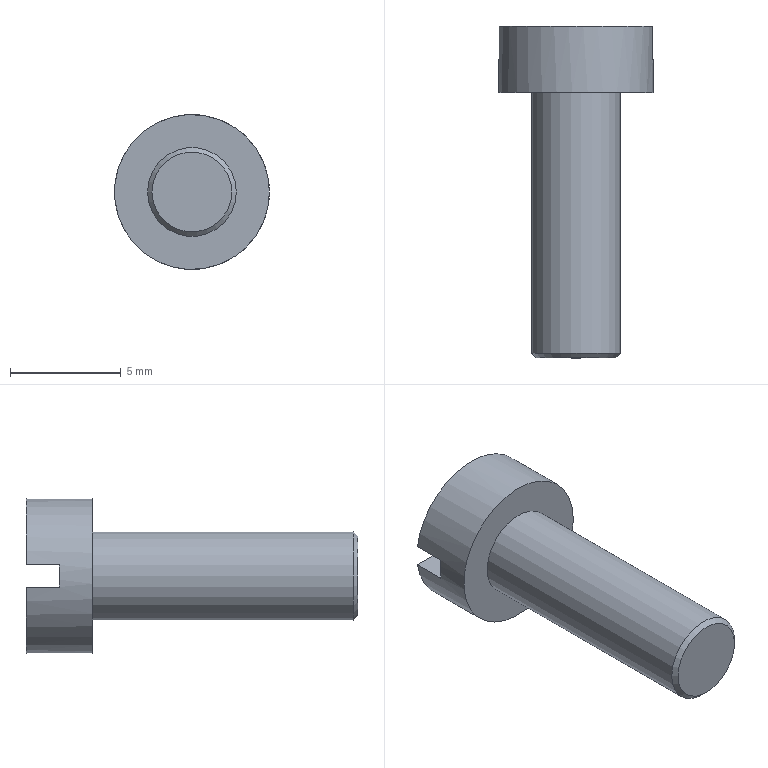Component | NX | SCREW_M4 | 1 solid | 10 faces | box 7 x 15 x 7 mm | volume 257 mm3 | plane 7 | cylinder 2 | cone 1 | commonest cylinder face diameters 7 x1 4.013 x1
STEP:
#1=CARTESIAN_POINT('',(0.,0.,0.));
#2=DIRECTION('',(0.,0.,1.));
#3=DIRECTION('',(1.,0.,0.));
#4=AXIS2_PLACEMENT_3D('',#1,#2,#3);
#5=CARTESIAN_POINT('',(23.036,8.,105.));
#6=VERTEX_POINT('',#5);
#7=CARTESIAN_POINT('',(29.964,8.,105.));
#8=VERTEX_POINT('',#7);
#9=CARTESIAN_POINT('',(26.5,8.,104.5));
#10=DIRECTION('',(0.,1.,0.));
#11=DIRECTION('',(1.,0.,0.));
#12=AXIS2_PLACEMENT_3D('',#9,#10,#11);
#13=CIRCLE('',#12,3.5);
#14=CARTESIAN_POINT('',(26.5,8.,104.5));
#15=DIRECTION('',(0.,1.,0.));
#16=DIRECTION('',(1.,0.,0.));
#17=AXIS2_PLACEMENT_3D('',#14,#15,#16);
#18=PLANE('',#17);
#19=CARTESIAN_POINT('',(0.,0.));
#20=DIRECTION('',(1.,0.));
#21=AXIS2_PLACEMENT_2D('',#19,#20);
#22=CIRCLE('',#21,3.5);
#23=(GEOMETRIC_REPRESENTATION_CONTEXT(2)PARAMETRIC_REPRESENTATION_CONTEXT()REPRESENTATION_CONTEXT('',''));
#24=DEFINITIONAL_REPRESENTATION('',(#22),#23);
#25=PCURVE('',#18,#24);
#26=CARTESIAN_POINT('',(26.5,5.,104.5));
#27=DIRECTION('',(0.,1.,0.));
#28=DIRECTION('',(1.,0.,0.));
#29=AXIS2_PLACEMENT_3D('',#26,#27,#28);
#30=CYLINDRICAL_SURFACE('',#29,3.5);
#31=CARTESIAN_POINT('',(0.,3.));
#32=DIRECTION('',(1.,0.));
#33=VECTOR('',#32,1.);
#34=LINE('',#31,#33);
#35=(GEOMETRIC_REPRESENTATION_CONTEXT(2)PARAMETRIC_REPRESENTATION_CONTEXT()REPRESENTATION_CONTEXT('',''));
#36=DEFINITIONAL_REPRESENTATION('',(#34),#35);
#37=PCURVE('',#30,#36);
#38=SURFACE_CURVE('',#13,(#25,#37),.PCURVE_S1.);
#39=EDGE_CURVE('',#6,#8,#38,.T.);
#40=ORIENTED_EDGE('',*,*,#39,.T.);
#41=CARTESIAN_POINT('',(30.786,8.,105.));
#42=DIRECTION('',(-1.,0.,0.));
#43=VECTOR('',#42,1.);
#44=LINE('',#41,#43);
#45=CARTESIAN_POINT('',(4.286,-0.5));
#46=DIRECTION('',(-1.,0.));
#47=VECTOR('',#46,1.);
#48=LINE('',#45,#47);
#49=(GEOMETRIC_REPRESENTATION_CONTEXT(2)PARAMETRIC_REPRESENTATION_CONTEXT()REPRESENTATION_CONTEXT('',''));
#50=DEFINITIONAL_REPRESENTATION('',(#48),#49);
#51=PCURVE('',#18,#50);
#52=CARTESIAN_POINT('',(30.786,6.5,105.));
#53=DIRECTION('',(0.,0.,-1.));
#54=DIRECTION('',(0.,1.,0.));
#55=AXIS2_PLACEMENT_3D('',#52,#53,#54);
#56=PLANE('',#55);
#57=CARTESIAN_POINT('',(1.5,0.));
#58=DIRECTION('',(0.,-1.));
#59=VECTOR('',#58,1.);
#60=LINE('',#57,#59);
#61=(GEOMETRIC_REPRESENTATION_CONTEXT(2)PARAMETRIC_REPRESENTATION_CONTEXT()REPRESENTATION_CONTEXT('',''));
#62=DEFINITIONAL_REPRESENTATION('',(#60),#61);
#63=PCURVE('',#56,#62);
#64=SURFACE_CURVE('',#44,(#51,#63),.PCURVE_S1.);
#65=EDGE_CURVE('',#8,#6,#64,.T.);
#66=ORIENTED_EDGE('',*,*,#65,.T.);
#67=EDGE_LOOP('',(#40,#66));
#68=FACE_BOUND('',#67,.T.);
#69=ADVANCED_FACE('',(#68),#18,.T.);
#70=CARTESIAN_POINT('',(29.964,8.,104.));
#71=VERTEX_POINT('',#70);
#72=CARTESIAN_POINT('',(23.036,8.,104.));
#73=VERTEX_POINT('',#72);
#74=CARTESIAN_POINT('',(26.5,8.,104.5));
#75=DIRECTION('',(0.,1.,0.));
#76=DIRECTION('',(1.,0.,0.));
#77=AXIS2_PLACEMENT_3D('',#74,#75,#76);
#78=CIRCLE('',#77,3.5);
#79=CARTESIAN_POINT('',(26.5,8.,104.5));
#80=DIRECTION('',(0.,1.,0.));
#81=DIRECTION('',(1.,0.,0.));
#82=AXIS2_PLACEMENT_3D('',#79,#80,#81);
#83=PLANE('',#82);
#84=CARTESIAN_POINT('',(0.,0.));
#85=DIRECTION('',(1.,0.));
#86=AXIS2_PLACEMENT_2D('',#84,#85);
#87=CIRCLE('',#86,3.5);
#88=(GEOMETRIC_REPRESENTATION_CONTEXT(2)PARAMETRIC_REPRESENTATION_CONTEXT()REPRESENTATION_CONTEXT('',''));
#89=DEFINITIONAL_REPRESENTATION('',(#87),#88);
#90=PCURVE('',#83,#89);
#91=CARTESIAN_POINT('',(0.,3.));
#92=DIRECTION('',(1.,0.));
#93=VECTOR('',#92,1.);
#94=LINE('',#91,#93);
#95=(GEOMETRIC_REPRESENTATION_CONTEXT(2)PARAMETRIC_REPRESENTATION_CONTEXT()REPRESENTATION_CONTEXT('',''));
#96=DEFINITIONAL_REPRESENTATION('',(#94),#95);
#97=PCURVE('',#30,#96);
#98=SURFACE_CURVE('',#78,(#90,#97),.PCURVE_S1.);
#99=EDGE_CURVE('',#71,#73,#98,.T.);
#100=ORIENTED_EDGE('',*,*,#99,.T.);
#101=CARTESIAN_POINT('',(22.214,8.,104.));
#102=DIRECTION('',(1.,0.,0.));
#103=VECTOR('',#102,1.);
#104=LINE('',#101,#103);
#105=CARTESIAN_POINT('',(-4.286,0.5));
#106=DIRECTION('',(1.,0.));
#107=VECTOR('',#106,1.);
#108=LINE('',#105,#107);
#109=(GEOMETRIC_REPRESENTATION_CONTEXT(2)PARAMETRIC_REPRESENTATION_CONTEXT()REPRESENTATION_CONTEXT('',''));
#110=DEFINITIONAL_REPRESENTATION('',(#108),#109);
#111=PCURVE('',#83,#110);
#112=CARTESIAN_POINT('',(22.214,6.5,104.));
#113=DIRECTION('',(0.,0.,1.));
#114=DIRECTION('',(0.,-1.,0.));
#115=AXIS2_PLACEMENT_3D('',#112,#113,#114);
#116=PLANE('',#115);
#117=CARTESIAN_POINT('',(-1.5,0.));
#118=DIRECTION('',(0.,1.));
#119=VECTOR('',#118,1.);
#120=LINE('',#117,#119);
#121=(GEOMETRIC_REPRESENTATION_CONTEXT(2)PARAMETRIC_REPRESENTATION_CONTEXT()REPRESENTATION_CONTEXT('',''));
#122=DEFINITIONAL_REPRESENTATION('',(#120),#121);
#123=PCURVE('',#116,#122);
#124=SURFACE_CURVE('',#104,(#111,#123),.PCURVE_S1.);
#125=EDGE_CURVE('',#73,#71,#124,.T.);
#126=ORIENTED_EDGE('',*,*,#125,.T.);
#127=EDGE_LOOP('',(#100,#126));
#128=FACE_BOUND('',#127,.T.);
#129=ADVANCED_FACE('',(#128),#83,.T.);
#130=CARTESIAN_POINT('',(30.,5.,104.5));
#131=VERTEX_POINT('',#130);
#132=CARTESIAN_POINT('',(26.5,5.,104.5));
#133=DIRECTION('',(0.,1.,0.));
#134=DIRECTION('',(1.,0.,0.));
#135=AXIS2_PLACEMENT_3D('',#132,#133,#134);
#136=CIRCLE('',#135,3.5);
#137=CARTESIAN_POINT('',(0.,0.));
#138=DIRECTION('',(1.,0.));
#139=VECTOR('',#138,1.);
#140=LINE('',#137,#139);
#141=(GEOMETRIC_REPRESENTATION_CONTEXT(2)PARAMETRIC_REPRESENTATION_CONTEXT()REPRESENTATION_CONTEXT('',''));
#142=DEFINITIONAL_REPRESENTATION('',(#140),#141);
#143=PCURVE('',#30,#142);
#144=CARTESIAN_POINT('',(26.5,5.,104.5));
#145=DIRECTION('',(0.,-1.,0.));
#146=DIRECTION('',(-1.,0.,0.));
#147=AXIS2_PLACEMENT_3D('',#144,#145,#146);
#148=PLANE('',#147);
#149=CARTESIAN_POINT('',(-3.5,0.));
#150=CARTESIAN_POINT('',(-3.5,6.062));
#151=CARTESIAN_POINT('',(1.75,3.031));
#152=CARTESIAN_POINT('',(7.,0.));
#153=CARTESIAN_POINT('',(1.75,-3.031));
#154=CARTESIAN_POINT('',(-3.5,-6.062));
#155=CARTESIAN_POINT('',(-3.5,0.));
#156=(BOUNDED_CURVE()B_SPLINE_CURVE(2,(#149,#150,#151,#152,#153,#154,#155),.UNSPECIFIED.,.T.,.F.)B_SPLINE_CURVE_WITH_KNOTS((1,2,2,2,2,1),(-2.094,0.,2.094,4.189,6.283,8.378),.UNSPECIFIED.)CURVE()GEOMETRIC_REPRESENTATION_ITEM()RATIONAL_B_SPLINE_CURVE((1.,0.5,1.,0.5,1.,0.5,1.))REPRESENTATION_ITEM(''));
#157=(GEOMETRIC_REPRESENTATION_CONTEXT(2)PARAMETRIC_REPRESENTATION_CONTEXT()REPRESENTATION_CONTEXT('',''));
#158=DEFINITIONAL_REPRESENTATION('',(#156),#157);
#159=PCURVE('',#148,#158);
#160=SURFACE_CURVE('',#136,(#143,#159),.PCURVE_S1.);
#161=EDGE_CURVE('',#131,#131,#160,.T.);
#162=ORIENTED_EDGE('',*,*,#161,.T.);
#163=CARTESIAN_POINT('',(30.,6.5,104.5));
#164=VERTEX_POINT('',#163);
#165=CARTESIAN_POINT('',(30.,5.,104.5));
#166=CARTESIAN_POINT('',(30.,6.5,104.5));
#167=B_SPLINE_CURVE_WITH_KNOTS('',1,(#165,#166),.UNSPECIFIED.,.F.,.F.,(2,2),(0.,1.5),.PIECEWISE_BEZIER_KNOTS.);
#168=CARTESIAN_POINT('',(6.283,0.));
#169=DIRECTION('',(0.,1.));
#170=VECTOR('',#169,1.);
#171=LINE('',#168,#170);
#172=(GEOMETRIC_REPRESENTATION_CONTEXT(2)PARAMETRIC_REPRESENTATION_CONTEXT()REPRESENTATION_CONTEXT('',''));
#173=DEFINITIONAL_REPRESENTATION('',(#171),#172);
#174=PCURVE('',#30,#173);
#175=CARTESIAN_POINT('',(0.,0.));
#176=DIRECTION('',(0.,1.));
#177=VECTOR('',#176,1.);
#178=LINE('',#175,#177);
#179=(GEOMETRIC_REPRESENTATION_CONTEXT(2)PARAMETRIC_REPRESENTATION_CONTEXT()REPRESENTATION_CONTEXT('',''));
#180=DEFINITIONAL_REPRESENTATION('',(#178),#179);
#181=PCURVE('',#30,#180);
#182=SEAM_CURVE('',#167,(#174,#181),.PCURVE_S1.);
#183=EDGE_CURVE('',#131,#164,#182,.T.);
#184=ORIENTED_EDGE('',*,*,#183,.T.);
#185=CARTESIAN_POINT('',(29.964,6.5,105.));
#186=VERTEX_POINT('',#185);
#187=CARTESIAN_POINT('',(26.5,6.5,104.5));
#188=DIRECTION('',(0.,1.,0.));
#189=DIRECTION('',(-1.,0.,0.));
#190=AXIS2_PLACEMENT_3D('',#187,#188,#189);
#191=CIRCLE('',#190,3.5);
#192=CARTESIAN_POINT('',(3.142,1.5));
#193=DIRECTION('',(1.,0.));
#194=VECTOR('',#193,1.);
#195=LINE('',#192,#194);
#196=(GEOMETRIC_REPRESENTATION_CONTEXT(2)PARAMETRIC_REPRESENTATION_CONTEXT()REPRESENTATION_CONTEXT('',''));
#197=DEFINITIONAL_REPRESENTATION('',(#195),#196);
#198=PCURVE('',#30,#197);
#199=CARTESIAN_POINT('',(26.5,6.5,104.5));
#200=DIRECTION('',(0.,-1.,0.));
#201=DIRECTION('',(-1.,0.,0.));
#202=AXIS2_PLACEMENT_3D('',#199,#200,#201);
#203=PLANE('',#202);
#204=CARTESIAN_POINT('',(3.5,0.));
#205=CARTESIAN_POINT('',(3.5,-6.062));
#206=CARTESIAN_POINT('',(-1.75,-3.031));
#207=CARTESIAN_POINT('',(-7.,-0.));
#208=CARTESIAN_POINT('',(-1.75,3.031));
#209=CARTESIAN_POINT('',(3.5,6.062));
#210=CARTESIAN_POINT('',(3.5,0.));
#211=(BOUNDED_CURVE()B_SPLINE_CURVE(2,(#204,#205,#206,#207,#208,#209,#210),.UNSPECIFIED.,.T.,.F.)B_SPLINE_CURVE_WITH_KNOTS((1,2,2,2,2,1),(-2.094,0.,2.094,4.189,6.283,8.378),.UNSPECIFIED.)CURVE()GEOMETRIC_REPRESENTATION_ITEM()RATIONAL_B_SPLINE_CURVE((1.,0.5,1.,0.5,1.,0.5,1.))REPRESENTATION_ITEM(''));
#212=(GEOMETRIC_REPRESENTATION_CONTEXT(2)PARAMETRIC_REPRESENTATION_CONTEXT()REPRESENTATION_CONTEXT('',''));
#213=DEFINITIONAL_REPRESENTATION('',(#211),#212);
#214=PCURVE('',#203,#213);
#215=SURFACE_CURVE('',#191,(#198,#214),.PCURVE_S1.);
#216=EDGE_CURVE('',#186,#164,#215,.T.);
#217=ORIENTED_EDGE('',*,*,#216,.F.);
#218=CARTESIAN_POINT('',(29.964,5.,105.));
#219=DIRECTION('',(0.,1.,0.));
#220=VECTOR('',#219,1.);
#221=LINE('',#218,#220);
#222=CARTESIAN_POINT('',(6.14,0.));
#223=DIRECTION('',(0.,1.));
#224=VECTOR('',#223,1.);
#225=LINE('',#222,#224);
#226=(GEOMETRIC_REPRESENTATION_CONTEXT(2)PARAMETRIC_REPRESENTATION_CONTEXT()REPRESENTATION_CONTEXT('',''));
#227=DEFINITIONAL_REPRESENTATION('',(#225),#226);
#228=PCURVE('',#30,#227);
#229=CARTESIAN_POINT('',(-1.5,-0.822));
#230=DIRECTION('',(1.,0.));
#231=VECTOR('',#230,1.);
#232=LINE('',#229,#231);
#233=(GEOMETRIC_REPRESENTATION_CONTEXT(2)PARAMETRIC_REPRESENTATION_CONTEXT()REPRESENTATION_CONTEXT('',''));
#234=DEFINITIONAL_REPRESENTATION('',(#232),#233);
#235=PCURVE('',#56,#234);
#236=SURFACE_CURVE('',#221,(#228,#235),.PCURVE_S1.);
#237=EDGE_CURVE('',#186,#8,#236,.T.);
#238=ORIENTED_EDGE('',*,*,#237,.T.);
#239=ORIENTED_EDGE('',*,*,#39,.F.);
#240=CARTESIAN_POINT('',(23.036,6.5,105.));
#241=VERTEX_POINT('',#240);
#242=CARTESIAN_POINT('',(23.036,5.,105.));
#243=DIRECTION('',(0.,-1.,0.));
#244=VECTOR('',#243,1.);
#245=LINE('',#242,#244);
#246=CARTESIAN_POINT('',(3.285,0.));
#247=DIRECTION('',(0.,-1.));
#248=VECTOR('',#247,1.);
#249=LINE('',#246,#248);
#250=(GEOMETRIC_REPRESENTATION_CONTEXT(2)PARAMETRIC_REPRESENTATION_CONTEXT()REPRESENTATION_CONTEXT('',''));
#251=DEFINITIONAL_REPRESENTATION('',(#249),#250);
#252=PCURVE('',#30,#251);
#253=CARTESIAN_POINT('',(-1.5,-7.75));
#254=DIRECTION('',(-1.,0.));
#255=VECTOR('',#254,1.);
#256=LINE('',#253,#255);
#257=(GEOMETRIC_REPRESENTATION_CONTEXT(2)PARAMETRIC_REPRESENTATION_CONTEXT()REPRESENTATION_CONTEXT('',''));
#258=DEFINITIONAL_REPRESENTATION('',(#256),#257);
#259=PCURVE('',#56,#258);
#260=SURFACE_CURVE('',#245,(#252,#259),.PCURVE_S1.);
#261=EDGE_CURVE('',#6,#241,#260,.T.);
#262=ORIENTED_EDGE('',*,*,#261,.T.);
#263=CARTESIAN_POINT('',(23.036,6.5,104.));
#264=VERTEX_POINT('',#263);
#265=CARTESIAN_POINT('',(26.5,6.5,104.5));
#266=DIRECTION('',(0.,1.,0.));
#267=DIRECTION('',(-1.,0.,0.));
#268=AXIS2_PLACEMENT_3D('',#265,#266,#267);
#269=CIRCLE('',#268,3.5);
#270=CARTESIAN_POINT('',(-3.142,1.5));
#271=DIRECTION('',(1.,0.));
#272=VECTOR('',#271,1.);
#273=LINE('',#270,#272);
#274=(GEOMETRIC_REPRESENTATION_CONTEXT(2)PARAMETRIC_REPRESENTATION_CONTEXT()REPRESENTATION_CONTEXT('',''));
#275=DEFINITIONAL_REPRESENTATION('',(#273),#274);
#276=PCURVE('',#30,#275);
#277=CARTESIAN_POINT('',(3.5,0.));
#278=CARTESIAN_POINT('',(3.5,-6.062));
#279=CARTESIAN_POINT('',(-1.75,-3.031));
#280=CARTESIAN_POINT('',(-7.,-0.));
#281=CARTESIAN_POINT('',(-1.75,3.031));
#282=CARTESIAN_POINT('',(3.5,6.062));
#283=CARTESIAN_POINT('',(3.5,0.));
#284=(BOUNDED_CURVE()B_SPLINE_CURVE(2,(#277,#278,#279,#280,#281,#282,#283),.UNSPECIFIED.,.T.,.F.)B_SPLINE_CURVE_WITH_KNOTS((1,2,2,2,2,1),(-2.094,0.,2.094,4.189,6.283,8.378),.UNSPECIFIED.)CURVE()GEOMETRIC_REPRESENTATION_ITEM()RATIONAL_B_SPLINE_CURVE((1.,0.5,1.,0.5,1.,0.5,1.))REPRESENTATION_ITEM(''));
#285=(GEOMETRIC_REPRESENTATION_CONTEXT(2)PARAMETRIC_REPRESENTATION_CONTEXT()REPRESENTATION_CONTEXT('',''));
#286=DEFINITIONAL_REPRESENTATION('',(#284),#285);
#287=PCURVE('',#203,#286);
#288=SURFACE_CURVE('',#269,(#276,#287),.PCURVE_S1.);
#289=EDGE_CURVE('',#264,#241,#288,.T.);
#290=ORIENTED_EDGE('',*,*,#289,.F.);
#291=CARTESIAN_POINT('',(23.036,5.,104.));
#292=DIRECTION('',(0.,1.,0.));
#293=VECTOR('',#292,1.);
#294=LINE('',#291,#293);
#295=CARTESIAN_POINT('',(2.998,0.));
#296=DIRECTION('',(0.,1.));
#297=VECTOR('',#296,1.);
#298=LINE('',#295,#297);
#299=(GEOMETRIC_REPRESENTATION_CONTEXT(2)PARAMETRIC_REPRESENTATION_CONTEXT()REPRESENTATION_CONTEXT('',''));
#300=DEFINITIONAL_REPRESENTATION('',(#298),#299);
#301=PCURVE('',#30,#300);
#302=CARTESIAN_POINT('',(1.5,0.822));
#303=DIRECTION('',(-1.,0.));
#304=VECTOR('',#303,1.);
#305=LINE('',#302,#304);
#306=(GEOMETRIC_REPRESENTATION_CONTEXT(2)PARAMETRIC_REPRESENTATION_CONTEXT()REPRESENTATION_CONTEXT('',''));
#307=DEFINITIONAL_REPRESENTATION('',(#305),#306);
#308=PCURVE('',#116,#307);
#309=SURFACE_CURVE('',#294,(#301,#308),.PCURVE_S1.);
#310=EDGE_CURVE('',#264,#73,#309,.T.);
#311=ORIENTED_EDGE('',*,*,#310,.T.);
#312=ORIENTED_EDGE('',*,*,#99,.F.);
#313=CARTESIAN_POINT('',(29.964,6.5,104.));
#314=VERTEX_POINT('',#313);
#315=CARTESIAN_POINT('',(29.964,5.,104.));
#316=DIRECTION('',(0.,-1.,0.));
#317=VECTOR('',#316,1.);
#318=LINE('',#315,#317);
#319=CARTESIAN_POINT('',(0.1433,0.));
#320=DIRECTION('',(0.,-1.));
#321=VECTOR('',#320,1.);
#322=LINE('',#319,#321);
#323=(GEOMETRIC_REPRESENTATION_CONTEXT(2)PARAMETRIC_REPRESENTATION_CONTEXT()REPRESENTATION_CONTEXT('',''));
#324=DEFINITIONAL_REPRESENTATION('',(#322),#323);
#325=PCURVE('',#30,#324);
#326=CARTESIAN_POINT('',(1.5,7.75));
#327=DIRECTION('',(1.,0.));
#328=VECTOR('',#327,1.);
#329=LINE('',#326,#328);
#330=(GEOMETRIC_REPRESENTATION_CONTEXT(2)PARAMETRIC_REPRESENTATION_CONTEXT()REPRESENTATION_CONTEXT('',''));
#331=DEFINITIONAL_REPRESENTATION('',(#329),#330);
#332=PCURVE('',#116,#331);
#333=SURFACE_CURVE('',#318,(#325,#332),.PCURVE_S1.);
#334=EDGE_CURVE('',#71,#314,#333,.T.);
#335=ORIENTED_EDGE('',*,*,#334,.T.);
#336=CARTESIAN_POINT('',(26.5,6.5,104.5));
#337=DIRECTION('',(0.,1.,0.));
#338=DIRECTION('',(-1.,0.,0.));
#339=AXIS2_PLACEMENT_3D('',#336,#337,#338);
#340=CIRCLE('',#339,3.5);
#341=CARTESIAN_POINT('',(-3.142,1.5));
#342=DIRECTION('',(1.,0.));
#343=VECTOR('',#342,1.);
#344=LINE('',#341,#343);
#345=(GEOMETRIC_REPRESENTATION_CONTEXT(2)PARAMETRIC_REPRESENTATION_CONTEXT()REPRESENTATION_CONTEXT('',''));
#346=DEFINITIONAL_REPRESENTATION('',(#344),#345);
#347=PCURVE('',#30,#346);
#348=CARTESIAN_POINT('',(3.5,0.));
#349=CARTESIAN_POINT('',(3.5,-6.062));
#350=CARTESIAN_POINT('',(-1.75,-3.031));
#351=CARTESIAN_POINT('',(-7.,-0.));
#352=CARTESIAN_POINT('',(-1.75,3.031));
#353=CARTESIAN_POINT('',(3.5,6.062));
#354=CARTESIAN_POINT('',(3.5,0.));
#355=(BOUNDED_CURVE()B_SPLINE_CURVE(2,(#348,#349,#350,#351,#352,#353,#354),.UNSPECIFIED.,.T.,.F.)B_SPLINE_CURVE_WITH_KNOTS((1,2,2,2,2,1),(-2.094,0.,2.094,4.189,6.283,8.378),.UNSPECIFIED.)CURVE()GEOMETRIC_REPRESENTATION_ITEM()RATIONAL_B_SPLINE_CURVE((1.,0.5,1.,0.5,1.,0.5,1.))REPRESENTATION_ITEM(''));
#356=(GEOMETRIC_REPRESENTATION_CONTEXT(2)PARAMETRIC_REPRESENTATION_CONTEXT()REPRESENTATION_CONTEXT('',''));
#357=DEFINITIONAL_REPRESENTATION('',(#355),#356);
#358=PCURVE('',#203,#357);
#359=SURFACE_CURVE('',#340,(#347,#358),.PCURVE_S1.);
#360=EDGE_CURVE('',#164,#314,#359,.T.);
#361=ORIENTED_EDGE('',*,*,#360,.F.);
#362=ORIENTED_EDGE('',*,*,#183,.F.);
#363=EDGE_LOOP('',(#162,#184,#217,#238,#239,#262,#290,#311,#312,#335,#361,#362));
#364=FACE_BOUND('',#363,.T.);
#365=ADVANCED_FACE('',(#364),#30,.T.);
#366=CARTESIAN_POINT('',(24.693,-7.,104.5));
#367=VERTEX_POINT('',#366);
#368=CARTESIAN_POINT('',(26.5,-7.,104.5));
#369=DIRECTION('',(0.,-1.,0.));
#370=DIRECTION('',(-1.,0.,0.));
#371=AXIS2_PLACEMENT_3D('',#368,#369,#370);
#372=CIRCLE('',#371,1.807);
#373=CARTESIAN_POINT('',(26.5,-7.,104.5));
#374=DIRECTION('',(0.,-1.,0.));
#375=DIRECTION('',(-1.,0.,0.));
#376=AXIS2_PLACEMENT_3D('',#373,#374,#375);
#377=PLANE('',#376);
#378=CARTESIAN_POINT('',(0.,0.));
#379=DIRECTION('',(1.,0.));
#380=AXIS2_PLACEMENT_2D('',#378,#379);
#381=CIRCLE('',#380,1.807);
#382=(GEOMETRIC_REPRESENTATION_CONTEXT(2)PARAMETRIC_REPRESENTATION_CONTEXT()REPRESENTATION_CONTEXT('',''));
#383=DEFINITIONAL_REPRESENTATION('',(#381),#382);
#384=PCURVE('',#377,#383);
#385=CARTESIAN_POINT('',(26.5,-6.8,104.5));
#386=DIRECTION('',(0.,1.,0.));
#387=DIRECTION('',(1.,0.,0.));
#388=AXIS2_PLACEMENT_3D('',#385,#386,#387);
#389=CONICAL_SURFACE('',#388,2.007,0.7854);
#390=CARTESIAN_POINT('',(9.425,-0.2));
#391=DIRECTION('',(-1.,0.));
#392=VECTOR('',#391,1.);
#393=LINE('',#390,#392);
#394=(GEOMETRIC_REPRESENTATION_CONTEXT(2)PARAMETRIC_REPRESENTATION_CONTEXT()REPRESENTATION_CONTEXT('',''));
#395=DEFINITIONAL_REPRESENTATION('',(#393),#394);
#396=PCURVE('',#389,#395);
#397=SURFACE_CURVE('',#372,(#384,#396),.PCURVE_S1.);
#398=EDGE_CURVE('',#367,#367,#397,.T.);
#399=ORIENTED_EDGE('',*,*,#398,.T.);
#400=EDGE_LOOP('',(#399));
#401=FACE_BOUND('',#400,.T.);
#402=ADVANCED_FACE('',(#401),#377,.T.);
#403=CARTESIAN_POINT('',(24.493,-6.8,104.5));
#404=VERTEX_POINT('',#403);
#405=CARTESIAN_POINT('',(28.507,-6.8,104.5));
#406=VERTEX_POINT('',#405);
#407=CARTESIAN_POINT('',(26.5,-6.8,104.5));
#408=DIRECTION('',(0.,1.,0.));
#409=DIRECTION('',(-1.,0.,0.));
#410=AXIS2_PLACEMENT_3D('',#407,#408,#409);
#411=CIRCLE('',#410,2.007);
#412=CARTESIAN_POINT('',(26.5,-7.,104.5));
#413=DIRECTION('',(0.,1.,0.));
#414=DIRECTION('',(1.,0.,0.));
#415=AXIS2_PLACEMENT_3D('',#412,#413,#414);
#416=CYLINDRICAL_SURFACE('',#415,2.007);
#417=CARTESIAN_POINT('',(3.142,0.2));
#418=DIRECTION('',(1.,0.));
#419=VECTOR('',#418,1.);
#420=LINE('',#417,#419);
#421=(GEOMETRIC_REPRESENTATION_CONTEXT(2)PARAMETRIC_REPRESENTATION_CONTEXT()REPRESENTATION_CONTEXT('',''));
#422=DEFINITIONAL_REPRESENTATION('',(#420),#421);
#423=PCURVE('',#416,#422);
#424=CARTESIAN_POINT('',(3.142,-0.));
#425=DIRECTION('',(1.,0.));
#426=VECTOR('',#425,1.);
#427=LINE('',#424,#426);
#428=(GEOMETRIC_REPRESENTATION_CONTEXT(2)PARAMETRIC_REPRESENTATION_CONTEXT()REPRESENTATION_CONTEXT('',''));
#429=DEFINITIONAL_REPRESENTATION('',(#427),#428);
#430=PCURVE('',#389,#429);
#431=SURFACE_CURVE('',#411,(#423,#430),.PCURVE_S1.);
#432=EDGE_CURVE('',#404,#406,#431,.T.);
#433=ORIENTED_EDGE('',*,*,#432,.T.);
#434=CARTESIAN_POINT('',(28.507,5.,104.5));
#435=VERTEX_POINT('',#434);
#436=CARTESIAN_POINT('',(28.507,-6.8,104.5));
#437=CARTESIAN_POINT('',(28.507,5.,104.5));
#438=B_SPLINE_CURVE_WITH_KNOTS('',1,(#436,#437),.UNSPECIFIED.,.F.,.F.,(2,2),(0.2,12.),.PIECEWISE_BEZIER_KNOTS.);
#439=CARTESIAN_POINT('',(6.283,0.));
#440=DIRECTION('',(0.,1.));
#441=VECTOR('',#440,1.);
#442=LINE('',#439,#441);
#443=(GEOMETRIC_REPRESENTATION_CONTEXT(2)PARAMETRIC_REPRESENTATION_CONTEXT()REPRESENTATION_CONTEXT('',''));
#444=DEFINITIONAL_REPRESENTATION('',(#442),#443);
#445=PCURVE('',#416,#444);
#446=CARTESIAN_POINT('',(0.,0.));
#447=DIRECTION('',(0.,1.));
#448=VECTOR('',#447,1.);
#449=LINE('',#446,#448);
#450=(GEOMETRIC_REPRESENTATION_CONTEXT(2)PARAMETRIC_REPRESENTATION_CONTEXT()REPRESENTATION_CONTEXT('',''));
#451=DEFINITIONAL_REPRESENTATION('',(#449),#450);
#452=PCURVE('',#416,#451);
#453=SEAM_CURVE('',#438,(#445,#452),.PCURVE_S1.);
#454=EDGE_CURVE('',#406,#435,#453,.T.);
#455=ORIENTED_EDGE('',*,*,#454,.T.);
#456=CARTESIAN_POINT('',(26.5,5.,104.5));
#457=DIRECTION('',(0.,-1.,0.));
#458=DIRECTION('',(1.,0.,0.));
#459=AXIS2_PLACEMENT_3D('',#456,#457,#458);
#460=CIRCLE('',#459,2.007);
#461=CARTESIAN_POINT('',(6.283,12.));
#462=DIRECTION('',(-1.,0.));
#463=VECTOR('',#462,1.);
#464=LINE('',#461,#463);
#465=(GEOMETRIC_REPRESENTATION_CONTEXT(2)PARAMETRIC_REPRESENTATION_CONTEXT()REPRESENTATION_CONTEXT('',''));
#466=DEFINITIONAL_REPRESENTATION('',(#464),#465);
#467=PCURVE('',#416,#466);
#468=CARTESIAN_POINT('',(0.,0.));
#469=DIRECTION('',(-1.,0.));
#470=AXIS2_PLACEMENT_2D('',#468,#469);
#471=CIRCLE('',#470,2.007);
#472=(GEOMETRIC_REPRESENTATION_CONTEXT(2)PARAMETRIC_REPRESENTATION_CONTEXT()REPRESENTATION_CONTEXT('',''));
#473=DEFINITIONAL_REPRESENTATION('',(#471),#472);
#474=PCURVE('',#148,#473);
#475=SURFACE_CURVE('',#460,(#467,#474),.PCURVE_S1.);
#476=EDGE_CURVE('',#435,#435,#475,.T.);
#477=ORIENTED_EDGE('',*,*,#476,.T.);
#478=ORIENTED_EDGE('',*,*,#454,.F.);
#479=CARTESIAN_POINT('',(26.5,-6.8,104.5));
#480=DIRECTION('',(0.,1.,0.));
#481=DIRECTION('',(-1.,0.,0.));
#482=AXIS2_PLACEMENT_3D('',#479,#480,#481);
#483=CIRCLE('',#482,2.007);
#484=CARTESIAN_POINT('',(-3.142,0.2));
#485=DIRECTION('',(1.,0.));
#486=VECTOR('',#485,1.);
#487=LINE('',#484,#486);
#488=(GEOMETRIC_REPRESENTATION_CONTEXT(2)PARAMETRIC_REPRESENTATION_CONTEXT()REPRESENTATION_CONTEXT('',''));
#489=DEFINITIONAL_REPRESENTATION('',(#487),#488);
#490=PCURVE('',#416,#489);
#491=CARTESIAN_POINT('',(3.142,-0.));
#492=DIRECTION('',(1.,0.));
#493=VECTOR('',#492,1.);
#494=LINE('',#491,#493);
#495=(GEOMETRIC_REPRESENTATION_CONTEXT(2)PARAMETRIC_REPRESENTATION_CONTEXT()REPRESENTATION_CONTEXT('',''));
#496=DEFINITIONAL_REPRESENTATION('',(#494),#495);
#497=PCURVE('',#389,#496);
#498=SURFACE_CURVE('',#483,(#490,#497),.PCURVE_S1.);
#499=EDGE_CURVE('',#406,#404,#498,.T.);
#500=ORIENTED_EDGE('',*,*,#499,.T.);
#501=EDGE_LOOP('',(#433,#455,#477,#478,#500));
#502=FACE_BOUND('',#501,.T.);
#503=ADVANCED_FACE('',(#502),#416,.T.);
#504=ORIENTED_EDGE('',*,*,#476,.F.);
#505=EDGE_LOOP('',(#504));
#506=FACE_BOUND('',#505,.T.);
#507=ORIENTED_EDGE('',*,*,#161,.F.);
#508=EDGE_LOOP('',(#507));
#509=FACE_BOUND('',#508,.T.);
#510=ADVANCED_FACE('',(#506,#509),#148,.T.);
#511=ORIENTED_EDGE('',*,*,#398,.F.);
#512=CARTESIAN_POINT('',(24.693,-7.,104.5));
#513=CARTESIAN_POINT('',(24.493,-6.8,104.5));
#514=B_SPLINE_CURVE_WITH_KNOTS('',1,(#512,#513),.UNSPECIFIED.,.F.,.F.,(2,2),(-0.2828,-0.),.PIECEWISE_BEZIER_KNOTS.);
#515=CARTESIAN_POINT('',(9.425,0.));
#516=DIRECTION('',(0.,1.));
#517=VECTOR('',#516,1.);
#518=LINE('',#515,#517);
#519=(GEOMETRIC_REPRESENTATION_CONTEXT(2)PARAMETRIC_REPRESENTATION_CONTEXT()REPRESENTATION_CONTEXT('',''));
#520=DEFINITIONAL_REPRESENTATION('',(#518),#519);
#521=PCURVE('',#389,#520);
#522=CARTESIAN_POINT('',(3.142,0.));
#523=DIRECTION('',(0.,1.));
#524=VECTOR('',#523,1.);
#525=LINE('',#522,#524);
#526=(GEOMETRIC_REPRESENTATION_CONTEXT(2)PARAMETRIC_REPRESENTATION_CONTEXT()REPRESENTATION_CONTEXT('',''));
#527=DEFINITIONAL_REPRESENTATION('',(#525),#526);
#528=PCURVE('',#389,#527);
#529=SEAM_CURVE('',#514,(#521,#528),.PCURVE_S1.);
#530=EDGE_CURVE('',#367,#404,#529,.T.);
#531=ORIENTED_EDGE('',*,*,#530,.T.);
#532=ORIENTED_EDGE('',*,*,#499,.F.);
#533=ORIENTED_EDGE('',*,*,#432,.F.);
#534=ORIENTED_EDGE('',*,*,#530,.F.);
#535=EDGE_LOOP('',(#511,#531,#532,#533,#534));
#536=FACE_BOUND('',#535,.T.);
#537=ADVANCED_FACE('',(#536),#389,.T.);
#538=ORIENTED_EDGE('',*,*,#65,.F.);
#539=ORIENTED_EDGE('',*,*,#237,.F.);
#540=CARTESIAN_POINT('',(30.786,6.5,105.));
#541=DIRECTION('',(1.,0.,0.));
#542=VECTOR('',#541,1.);
#543=LINE('',#540,#542);
#544=CARTESIAN_POINT('',(0.,0.));
#545=DIRECTION('',(0.,1.));
#546=VECTOR('',#545,1.);
#547=LINE('',#544,#546);
#548=(GEOMETRIC_REPRESENTATION_CONTEXT(2)PARAMETRIC_REPRESENTATION_CONTEXT()REPRESENTATION_CONTEXT('',''));
#549=DEFINITIONAL_REPRESENTATION('',(#547),#548);
#550=PCURVE('',#56,#549);
#551=CARTESIAN_POINT('',(-4.286,-0.5));
#552=DIRECTION('',(-1.,0.));
#553=VECTOR('',#552,1.);
#554=LINE('',#551,#553);
#555=(GEOMETRIC_REPRESENTATION_CONTEXT(2)PARAMETRIC_REPRESENTATION_CONTEXT()REPRESENTATION_CONTEXT('',''));
#556=DEFINITIONAL_REPRESENTATION('',(#554),#555);
#557=PCURVE('',#203,#556);
#558=SURFACE_CURVE('',#543,(#550,#557),.PCURVE_S1.);
#559=EDGE_CURVE('',#241,#186,#558,.T.);
#560=ORIENTED_EDGE('',*,*,#559,.F.);
#561=ORIENTED_EDGE('',*,*,#261,.F.);
#562=EDGE_LOOP('',(#538,#539,#560,#561));
#563=FACE_BOUND('',#562,.T.);
#564=ADVANCED_FACE('',(#563),#56,.T.);
#565=ORIENTED_EDGE('',*,*,#125,.F.);
#566=ORIENTED_EDGE('',*,*,#310,.F.);
#567=CARTESIAN_POINT('',(22.214,6.5,104.));
#568=DIRECTION('',(-1.,0.,0.));
#569=VECTOR('',#568,1.);
#570=LINE('',#567,#569);
#571=CARTESIAN_POINT('',(0.,0.));
#572=DIRECTION('',(0.,-1.));
#573=VECTOR('',#572,1.);
#574=LINE('',#571,#573);
#575=(GEOMETRIC_REPRESENTATION_CONTEXT(2)PARAMETRIC_REPRESENTATION_CONTEXT()REPRESENTATION_CONTEXT('',''));
#576=DEFINITIONAL_REPRESENTATION('',(#574),#575);
#577=PCURVE('',#116,#576);
#578=CARTESIAN_POINT('',(4.286,0.5));
#579=DIRECTION('',(1.,0.));
#580=VECTOR('',#579,1.);
#581=LINE('',#578,#580);
#582=(GEOMETRIC_REPRESENTATION_CONTEXT(2)PARAMETRIC_REPRESENTATION_CONTEXT()REPRESENTATION_CONTEXT('',''));
#583=DEFINITIONAL_REPRESENTATION('',(#581),#582);
#584=PCURVE('',#203,#583);
#585=SURFACE_CURVE('',#570,(#577,#584),.PCURVE_S1.);
#586=EDGE_CURVE('',#314,#264,#585,.T.);
#587=ORIENTED_EDGE('',*,*,#586,.F.);
#588=ORIENTED_EDGE('',*,*,#334,.F.);
#589=EDGE_LOOP('',(#565,#566,#587,#588));
#590=FACE_BOUND('',#589,.T.);
#591=ADVANCED_FACE('',(#590),#116,.T.);
#592=ORIENTED_EDGE('',*,*,#216,.T.);
#593=ORIENTED_EDGE('',*,*,#360,.T.);
#594=ORIENTED_EDGE('',*,*,#586,.T.);
#595=ORIENTED_EDGE('',*,*,#289,.T.);
#596=ORIENTED_EDGE('',*,*,#559,.T.);
#597=EDGE_LOOP('',(#592,#593,#594,#595,#596));
#598=FACE_BOUND('',#597,.T.);
#599=ADVANCED_FACE('',(#598),#203,.F.);
#600=CLOSED_SHELL('',(#69,#129,#365,#402,#503,#510,#537,#564,#591,#599));
#601=MANIFOLD_SOLID_BREP('',#600);
#602=(LENGTH_UNIT()NAMED_UNIT(*)SI_UNIT(.MILLI.,.METRE.));
#603=UNCERTAINTY_MEASURE_WITH_UNIT(LENGTH_MEASURE(0.000002),#602,'','');
#604=(NAMED_UNIT(*)PLANE_ANGLE_UNIT()SI_UNIT($,.RADIAN.));
#605=(NAMED_UNIT(*)SI_UNIT($,.STERADIAN.)SOLID_ANGLE_UNIT());
#606=(GEOMETRIC_REPRESENTATION_CONTEXT(3)GLOBAL_UNCERTAINTY_ASSIGNED_CONTEXT((#603))GLOBAL_UNIT_ASSIGNED_CONTEXT((#602,#604,#605))REPRESENTATION_CONTEXT('',''));
#607=ADVANCED_BREP_SHAPE_REPRESENTATION('',(#4,#601),#606);